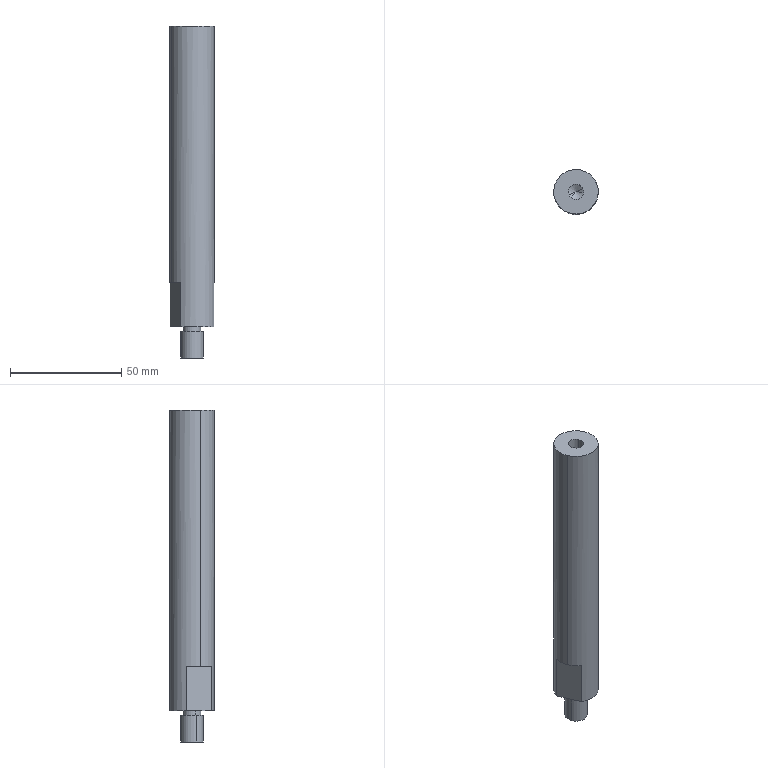Component | SolidWorks | -SmallSupport-2 | 1 solid | 18 faces | box 20 x 20 x 149 mm | volume 41968 mm3 | cylinder 8 | plane 8 | cone 2 | commonest cylinder face diameters 10 x2 8 x2 6.8 x2 20 x2
build123d program:
from build123d import *

# Parameters (mm, degrees)
SKETCH1_R             = 10
BOSS_EXTRUDE1_DEPTH   = 67.5
M8_TAPPED_HOLE1_D     = 6.8
M8_TAPPED_HOLE1_DEPTH = 22.25
M8_TAPPED_HOLE1_TIP   = 2.043
SKETCH4_R             = 4
BOSS_EXTRUDE2_DEPTH   = 2
SKETCH5_R             = 5
BOSS_EXTRUDE3_DEPTH   = 12
SKETCH6_W             = 8.326
SKETCH6_H             = 20.836
SKETCH6_W_2           = 8.024
SKETCH6_H_2           = 19.024
CUT_EXTRUDE1_DEPTH    = 20


with BuildPart() as part:
    # Sketch1 → Boss-Extrude1 (new, symmetric)
    with BuildSketch(Plane.XY):
        Circle(SKETCH1_R)
    extrude(amount=BOSS_EXTRUDE1_DEPTH, both=True)

    # M8 Tapped Hole1
    with Locations(Plane(origin=(0, 0, -67.5), x_dir=(1, 0, 0), z_dir=(0, 0, -1))):
        with Locations((0, 0)):
            Hole(M8_TAPPED_HOLE1_D / 2, depth=M8_TAPPED_HOLE1_DEPTH)
            with Locations((0, 0, -(M8_TAPPED_HOLE1_DEPTH + M8_TAPPED_HOLE1_TIP / 2))):  # 118° drill point
                Cone(0, M8_TAPPED_HOLE1_D / 2, M8_TAPPED_HOLE1_TIP, mode=Mode.SUBTRACT)

    # Sketch4 → Boss-Extrude2 (add)
    with BuildSketch(Plane.XY.offset(67.5)):
        Circle(SKETCH4_R)
    extrude(amount=BOSS_EXTRUDE2_DEPTH)

    # Sketch5 → Boss-Extrude3 (add)
    with BuildSketch(Plane.XY.offset(69.5)):
        Circle(SKETCH5_R)
    extrude(amount=BOSS_EXTRUDE3_DEPTH)

    # Sketch6 → Cut-Extrude1 (cut)
    with BuildSketch(Plane.XY.offset(67.5)):
        with Locations((-12.163, -0.5023)):
            Rectangle(SKETCH6_W, SKETCH6_H)
        with Locations((12.012, -1.408)):
            Rectangle(SKETCH6_W_2, SKETCH6_H_2)
    extrude(amount=-CUT_EXTRUDE1_DEPTH, mode=Mode.SUBTRACT)


solid = part.part

# Placed as in the assembly
solid = solid.moved(Location((115, 1079.5, 72.5), (-180, 0, 157.477)))
STEP:
#1=COLOUR_RGB('',0.7922,0.8196,0.9333);
#2=FILL_AREA_STYLE_COLOUR('',#1);
#3=FILL_AREA_STYLE('',(#2));
#4=SURFACE_STYLE_FILL_AREA(#3);
#5=SURFACE_SIDE_STYLE('',(#4));
#6=SURFACE_STYLE_USAGE(.BOTH.,#5);
#7=PRESENTATION_STYLE_ASSIGNMENT((#6));
#8=CARTESIAN_POINT('',(4.346,42.425,-0.3543));
#9=VERTEX_POINT('',#8);
#10=CARTESIAN_POINT('',(4.709,42.575,-0.3543));
#11=VERTEX_POINT('',#10);
#12=CARTESIAN_POINT('',(4.528,42.5,-0.3543));
#13=DIRECTION('',(0.,0.,-1.));
#14=DIRECTION('',(-0.9237,-0.383,0.));
#15=AXIS2_PLACEMENT_3D('',#12,#13,#14);
#16=CIRCLE('',#15,0.1969);
#17=EDGE_CURVE('',#9,#11,#16,.T.);
#18=ORIENTED_EDGE('',*,*,#17,.F.);
#19=CARTESIAN_POINT('',(4.346,42.425,0.1181));
#20=VERTEX_POINT('',#19);
#21=CARTESIAN_POINT('',(4.346,42.425,-0.3543));
#22=DIRECTION('',(0.,0.,1.));
#23=VECTOR('',#22,39.37);
#24=LINE('',#21,#23);
#25=EDGE_CURVE('',#9,#20,#24,.T.);
#26=ORIENTED_EDGE('',*,*,#25,.T.);
#27=CARTESIAN_POINT('',(4.709,42.575,0.1181));
#28=VERTEX_POINT('',#27);
#29=CARTESIAN_POINT('',(4.528,42.5,0.1181));
#30=DIRECTION('',(0.,0.,-1.));
#31=DIRECTION('',(-0.9237,-0.383,0.));
#32=AXIS2_PLACEMENT_3D('',#29,#30,#31);
#33=CIRCLE('',#32,0.1969);
#34=EDGE_CURVE('',#20,#28,#33,.T.);
#35=ORIENTED_EDGE('',*,*,#34,.T.);
#36=CARTESIAN_POINT('',(4.709,42.575,-0.3543));
#37=DIRECTION('',(0.,0.,1.));
#38=VECTOR('',#37,39.37);
#39=LINE('',#36,#38);
#40=EDGE_CURVE('',#11,#28,#39,.T.);
#41=ORIENTED_EDGE('',*,*,#40,.F.);
#42=EDGE_LOOP('',(#18,#26,#35,#41));
#43=FACE_OUTER_BOUND('',#42,.T.);
#44=CARTESIAN_POINT('',(4.528,42.5,-0.3543));
#45=DIRECTION('',(0.,0.,1.));
#46=DIRECTION('',(0.9237,0.383,0.));
#47=AXIS2_PLACEMENT_3D('',#44,#45,#46);
#48=CYLINDRICAL_SURFACE('',#47,0.1969);
#49=ADVANCED_FACE('',(#43),#48,.T.);
#50=CARTESIAN_POINT('',(4.382,42.44,0.1181));
#51=VERTEX_POINT('',#50);
#52=CARTESIAN_POINT('',(4.673,42.56,0.1181));
#53=VERTEX_POINT('',#52);
#54=CARTESIAN_POINT('',(4.528,42.5,0.1181));
#55=DIRECTION('',(0.,0.,-1.));
#56=DIRECTION('',(-0.9237,-0.383,0.));
#57=AXIS2_PLACEMENT_3D('',#54,#55,#56);
#58=CIRCLE('',#57,0.1575);
#59=EDGE_CURVE('',#51,#53,#58,.T.);
#60=ORIENTED_EDGE('',*,*,#59,.F.);
#61=CARTESIAN_POINT('',(4.382,42.44,0.1969));
#62=VERTEX_POINT('',#61);
#63=CARTESIAN_POINT('',(4.382,42.44,0.1181));
#64=DIRECTION('',(0.,0.,1.));
#65=VECTOR('',#64,39.37);
#66=LINE('',#63,#65);
#67=EDGE_CURVE('',#51,#62,#66,.T.);
#68=ORIENTED_EDGE('',*,*,#67,.T.);
#69=CARTESIAN_POINT('',(4.673,42.56,0.1969));
#70=VERTEX_POINT('',#69);
#71=CARTESIAN_POINT('',(4.528,42.5,0.1969));
#72=DIRECTION('',(0.,0.,-1.));
#73=DIRECTION('',(-0.9237,-0.383,0.));
#74=AXIS2_PLACEMENT_3D('',#71,#72,#73);
#75=CIRCLE('',#74,0.1575);
#76=EDGE_CURVE('',#62,#70,#75,.T.);
#77=ORIENTED_EDGE('',*,*,#76,.T.);
#78=CARTESIAN_POINT('',(4.673,42.56,0.1181));
#79=DIRECTION('',(0.,0.,1.));
#80=VECTOR('',#79,39.37);
#81=LINE('',#78,#80);
#82=EDGE_CURVE('',#53,#70,#81,.T.);
#83=ORIENTED_EDGE('',*,*,#82,.F.);
#84=EDGE_LOOP('',(#60,#68,#77,#83));
#85=FACE_OUTER_BOUND('',#84,.T.);
#86=CARTESIAN_POINT('',(4.528,42.5,0.1181));
#87=DIRECTION('',(0.,0.,1.));
#88=DIRECTION('',(0.9237,0.383,0.));
#89=AXIS2_PLACEMENT_3D('',#86,#87,#88);
#90=CYLINDRICAL_SURFACE('',#89,0.1575);
#91=ADVANCED_FACE('',(#85),#90,.T.);
#92=CARTESIAN_POINT('',(4.404,42.449,4.636));
#93=VERTEX_POINT('',#92);
#94=CARTESIAN_POINT('',(4.651,42.551,4.636));
#95=VERTEX_POINT('',#94);
#96=CARTESIAN_POINT('',(4.528,42.5,4.636));
#97=DIRECTION('',(0.,0.,1.));
#98=DIRECTION('',(0.9237,0.383,0.));
#99=AXIS2_PLACEMENT_3D('',#96,#97,#98);
#100=CIRCLE('',#99,0.1339);
#101=EDGE_CURVE('',#93,#95,#100,.T.);
#102=ORIENTED_EDGE('',*,*,#101,.F.);
#103=CARTESIAN_POINT('',(4.404,42.449,5.512));
#104=VERTEX_POINT('',#103);
#105=CARTESIAN_POINT('',(4.404,42.449,5.512));
#106=DIRECTION('',(0.,0.,1.));
#107=VECTOR('',#106,39.37);
#108=LINE('',#105,#107);
#109=EDGE_CURVE('',#93,#104,#108,.T.);
#110=ORIENTED_EDGE('',*,*,#109,.T.);
#111=CARTESIAN_POINT('',(4.651,42.551,5.512));
#112=VERTEX_POINT('',#111);
#113=CARTESIAN_POINT('',(4.528,42.5,5.512));
#114=DIRECTION('',(0.,0.,1.));
#115=DIRECTION('',(0.9237,0.383,0.));
#116=AXIS2_PLACEMENT_3D('',#113,#114,#115);
#117=CIRCLE('',#116,0.1339);
#118=EDGE_CURVE('',#104,#112,#117,.T.);
#119=ORIENTED_EDGE('',*,*,#118,.T.);
#120=CARTESIAN_POINT('',(4.651,42.551,5.512));
#121=DIRECTION('',(0.,0.,1.));
#122=VECTOR('',#121,39.37);
#123=LINE('',#120,#122);
#124=EDGE_CURVE('',#95,#112,#123,.T.);
#125=ORIENTED_EDGE('',*,*,#124,.F.);
#126=EDGE_LOOP('',(#102,#110,#119,#125));
#127=FACE_OUTER_BOUND('',#126,.T.);
#128=CARTESIAN_POINT('',(4.528,42.5,5.512));
#129=DIRECTION('',(0.,0.,1.));
#130=DIRECTION('',(0.9237,0.383,0.));
#131=AXIS2_PLACEMENT_3D('',#128,#129,#130);
#132=CYLINDRICAL_SURFACE('',#131,0.1339);
#133=ADVANCED_FACE('',(#127),#132,.F.);
#134=CARTESIAN_POINT('',(4.528,42.5,4.555));
#135=VERTEX_POINT('',#134);
#136=CARTESIAN_POINT('',(4.651,42.551,4.636));
#137=DIRECTION('',(0.7918,0.3283,0.515));
#138=VECTOR('',#137,39.37);
#139=LINE('',#136,#138);
#140=EDGE_CURVE('',#135,#95,#139,.T.);
#141=ORIENTED_EDGE('',*,*,#140,.F.);
#142=CARTESIAN_POINT('',(4.404,42.449,4.636));
#143=DIRECTION('',(-0.7918,-0.3283,0.515));
#144=VECTOR('',#143,39.37);
#145=LINE('',#142,#144);
#146=EDGE_CURVE('',#135,#93,#145,.T.);
#147=ORIENTED_EDGE('',*,*,#146,.T.);
#148=ORIENTED_EDGE('',*,*,#101,.T.);
#149=EDGE_LOOP('',(#141,#147,#148));
#150=FACE_OUTER_BOUND('',#149,.T.);
#151=CARTESIAN_POINT('',(4.528,42.5,4.636));
#152=DIRECTION('',(0.,0.,1.));
#153=DIRECTION('',(0.9237,0.383,0.));
#154=AXIS2_PLACEMENT_3D('',#151,#152,#153);
#155=CONICAL_SURFACE('',#154,0.1339,1.03);
#156=ADVANCED_FACE('',(#150),#155,.F.);
#157=CARTESIAN_POINT('',(4.146,42.598,0.9843));
#158=VERTEX_POINT('',#157);
#159=CARTESIAN_POINT('',(4.164,42.349,0.9843));
#160=VERTEX_POINT('',#159);
#161=CARTESIAN_POINT('',(4.528,42.5,0.9843));
#162=DIRECTION('',(0.,0.,1.));
#163=DIRECTION('',(0.9237,0.383,0.));
#164=AXIS2_PLACEMENT_3D('',#161,#162,#163);
#165=CIRCLE('',#164,0.3937);
#166=EDGE_CURVE('',#158,#160,#165,.T.);
#167=ORIENTED_EDGE('',*,*,#166,.T.);
#168=CARTESIAN_POINT('',(4.164,42.349,5.512));
#169=VERTEX_POINT('',#168);
#170=CARTESIAN_POINT('',(4.164,42.349,0.1969));
#171=DIRECTION('',(0.,0.,1.));
#172=VECTOR('',#171,39.37);
#173=LINE('',#170,#172);
#174=EDGE_CURVE('',#160,#169,#173,.T.);
#175=ORIENTED_EDGE('',*,*,#174,.T.);
#176=CARTESIAN_POINT('',(4.891,42.651,5.512));
#177=VERTEX_POINT('',#176);
#178=CARTESIAN_POINT('',(4.528,42.5,5.512));
#179=DIRECTION('',(0.,0.,-1.));
#180=DIRECTION('',(-0.9237,-0.383,0.));
#181=AXIS2_PLACEMENT_3D('',#178,#179,#180);
#182=CIRCLE('',#181,0.3937);
#183=EDGE_CURVE('',#169,#177,#182,.T.);
#184=ORIENTED_EDGE('',*,*,#183,.T.);
#185=CARTESIAN_POINT('',(4.891,42.651,0.9843));
#186=VERTEX_POINT('',#185);
#187=CARTESIAN_POINT('',(4.891,42.651,0.1969));
#188=DIRECTION('',(0.,0.,1.));
#189=VECTOR('',#188,39.37);
#190=LINE('',#187,#189);
#191=EDGE_CURVE('',#186,#177,#190,.T.);
#192=ORIENTED_EDGE('',*,*,#191,.F.);
#193=CARTESIAN_POINT('',(4.728,42.839,0.9843));
#194=VERTEX_POINT('',#193);
#195=CARTESIAN_POINT('',(4.528,42.5,0.9843));
#196=DIRECTION('',(0.,0.,-1.));
#197=DIRECTION('',(-0.9237,-0.383,0.));
#198=AXIS2_PLACEMENT_3D('',#195,#196,#197);
#199=CIRCLE('',#198,0.3937);
#200=EDGE_CURVE('',#194,#186,#199,.T.);
#201=ORIENTED_EDGE('',*,*,#200,.F.);
#202=CARTESIAN_POINT('',(4.728,42.839,0.1969));
#203=VERTEX_POINT('',#202);
#204=CARTESIAN_POINT('',(4.728,42.839,0.1969));
#205=DIRECTION('',(0.,0.,-1.));
#206=VECTOR('',#205,39.37);
#207=LINE('',#204,#206);
#208=EDGE_CURVE('',#194,#203,#207,.T.);
#209=ORIENTED_EDGE('',*,*,#208,.T.);
#210=CARTESIAN_POINT('',(4.146,42.598,0.1969));
#211=VERTEX_POINT('',#210);
#212=CARTESIAN_POINT('',(4.528,42.5,0.1969));
#213=DIRECTION('',(0.,0.,-1.));
#214=DIRECTION('',(-0.9237,-0.383,0.));
#215=AXIS2_PLACEMENT_3D('',#212,#213,#214);
#216=CIRCLE('',#215,0.3937);
#217=EDGE_CURVE('',#211,#203,#216,.T.);
#218=ORIENTED_EDGE('',*,*,#217,.F.);
#219=CARTESIAN_POINT('',(4.146,42.598,0.1969));
#220=DIRECTION('',(0.,0.,1.));
#221=VECTOR('',#220,39.37);
#222=LINE('',#219,#221);
#223=EDGE_CURVE('',#211,#158,#222,.T.);
#224=ORIENTED_EDGE('',*,*,#223,.T.);
#225=EDGE_LOOP('',(#167,#175,#184,#192,#201,#209,#218,#224));
#226=FACE_OUTER_BOUND('',#225,.T.);
#227=CARTESIAN_POINT('',(4.528,42.5,0.1969));
#228=DIRECTION('',(0.,0.,1.));
#229=DIRECTION('',(0.9237,0.383,0.));
#230=AXIS2_PLACEMENT_3D('',#227,#228,#229);
#231=CYLINDRICAL_SURFACE('',#230,0.3937);
#232=ADVANCED_FACE('',(#226),#231,.T.);
#233=CARTESIAN_POINT('',(4.327,42.161,0.1969));
#234=VERTEX_POINT('',#233);
#235=CARTESIAN_POINT('',(4.114,42.674,0.1969));
#236=DIRECTION('',(0.383,-0.9237,0.));
#237=VECTOR('',#236,39.37);
#238=LINE('',#235,#237);
#239=EDGE_CURVE('',#211,#234,#238,.T.);
#240=ORIENTED_EDGE('',*,*,#239,.F.);
#241=ORIENTED_EDGE('',*,*,#217,.T.);
#242=CARTESIAN_POINT('',(4.909,42.402,0.1969));
#243=VERTEX_POINT('',#242);
#244=CARTESIAN_POINT('',(4.669,42.981,0.1969));
#245=DIRECTION('',(-0.383,0.9237,0.));
#246=VECTOR('',#245,39.37);
#247=LINE('',#244,#246);
#248=EDGE_CURVE('',#243,#203,#247,.T.);
#249=ORIENTED_EDGE('',*,*,#248,.F.);
#250=CARTESIAN_POINT('',(4.528,42.5,0.1969));
#251=DIRECTION('',(0.,0.,-1.));
#252=DIRECTION('',(-0.9237,-0.383,0.));
#253=AXIS2_PLACEMENT_3D('',#250,#251,#252);
#254=CIRCLE('',#253,0.3937);
#255=EDGE_CURVE('',#243,#234,#254,.T.);
#256=ORIENTED_EDGE('',*,*,#255,.T.);
#257=EDGE_LOOP('',(#240,#241,#249,#256));
#258=FACE_OUTER_BOUND('',#257,.T.);
#259=CARTESIAN_POINT('',(4.528,42.5,0.1969));
#260=DIRECTION('',(0.,0.,-1.));
#261=DIRECTION('',(-0.9237,-0.383,0.));
#262=AXIS2_PLACEMENT_3D('',#259,#260,#261);
#263=CIRCLE('',#262,0.1575);
#264=EDGE_CURVE('',#70,#62,#263,.T.);
#265=ORIENTED_EDGE('',*,*,#264,.F.);
#266=ORIENTED_EDGE('',*,*,#76,.F.);
#267=EDGE_LOOP('',(#265,#266));
#268=FACE_BOUND('',#267,.T.);
#269=CARTESIAN_POINT('',(4.528,42.5,0.1969));
#270=DIRECTION('',(0.,0.,-1.));
#271=DIRECTION('',(-0.9237,-0.383,0.));
#272=AXIS2_PLACEMENT_3D('',#269,#270,#271);
#273=PLANE('',#272);
#274=ADVANCED_FACE('',(#258,#268),#273,.T.);
#275=ORIENTED_EDGE('',*,*,#174,.F.);
#276=CARTESIAN_POINT('',(4.327,42.161,0.9843));
#277=VERTEX_POINT('',#276);
#278=CARTESIAN_POINT('',(4.528,42.5,0.9843));
#279=DIRECTION('',(0.,0.,1.));
#280=DIRECTION('',(0.9237,0.383,0.));
#281=AXIS2_PLACEMENT_3D('',#278,#279,#280);
#282=CIRCLE('',#281,0.3937);
#283=EDGE_CURVE('',#160,#277,#282,.T.);
#284=ORIENTED_EDGE('',*,*,#283,.T.);
#285=CARTESIAN_POINT('',(4.327,42.161,0.1969));
#286=DIRECTION('',(0.,0.,-1.));
#287=VECTOR('',#286,39.37);
#288=LINE('',#285,#287);
#289=EDGE_CURVE('',#277,#234,#288,.T.);
#290=ORIENTED_EDGE('',*,*,#289,.T.);
#291=ORIENTED_EDGE('',*,*,#255,.F.);
#292=CARTESIAN_POINT('',(4.909,42.402,0.9843));
#293=VERTEX_POINT('',#292);
#294=CARTESIAN_POINT('',(4.909,42.402,0.1969));
#295=DIRECTION('',(0.,0.,1.));
#296=VECTOR('',#295,39.37);
#297=LINE('',#294,#296);
#298=EDGE_CURVE('',#243,#293,#297,.T.);
#299=ORIENTED_EDGE('',*,*,#298,.T.);
#300=CARTESIAN_POINT('',(4.528,42.5,0.9843));
#301=DIRECTION('',(0.,0.,-1.));
#302=DIRECTION('',(-0.9237,-0.383,0.));
#303=AXIS2_PLACEMENT_3D('',#300,#301,#302);
#304=CIRCLE('',#303,0.3937);
#305=EDGE_CURVE('',#186,#293,#304,.T.);
#306=ORIENTED_EDGE('',*,*,#305,.F.);
#307=ORIENTED_EDGE('',*,*,#191,.T.);
#308=CARTESIAN_POINT('',(4.528,42.5,5.512));
#309=DIRECTION('',(0.,0.,-1.));
#310=DIRECTION('',(-0.9237,-0.383,0.));
#311=AXIS2_PLACEMENT_3D('',#308,#309,#310);
#312=CIRCLE('',#311,0.3937);
#313=EDGE_CURVE('',#177,#169,#312,.T.);
#314=ORIENTED_EDGE('',*,*,#313,.T.);
#315=EDGE_LOOP('',(#275,#284,#290,#291,#299,#306,#307,#314));
#316=FACE_OUTER_BOUND('',#315,.T.);
#317=CARTESIAN_POINT('',(4.528,42.5,0.1969));
#318=DIRECTION('',(0.,0.,1.));
#319=DIRECTION('',(0.9237,0.383,0.));
#320=AXIS2_PLACEMENT_3D('',#317,#318,#319);
#321=CYLINDRICAL_SURFACE('',#320,0.3937);
#322=ADVANCED_FACE('',(#316),#321,.T.);
#323=CARTESIAN_POINT('',(4.528,42.5,5.512));
#324=DIRECTION('',(0.,0.,1.));
#325=DIRECTION('',(0.9237,0.383,0.));
#326=AXIS2_PLACEMENT_3D('',#323,#324,#325);
#327=CIRCLE('',#326,0.1339);
#328=EDGE_CURVE('',#112,#104,#327,.T.);
#329=ORIENTED_EDGE('',*,*,#328,.F.);
#330=ORIENTED_EDGE('',*,*,#118,.F.);
#331=EDGE_LOOP('',(#329,#330));
#332=FACE_BOUND('',#331,.T.);
#333=ORIENTED_EDGE('',*,*,#313,.F.);
#334=ORIENTED_EDGE('',*,*,#183,.F.);
#335=EDGE_LOOP('',(#333,#334));
#336=FACE_OUTER_BOUND('',#335,.T.);
#337=CARTESIAN_POINT('',(4.528,42.5,5.512));
#338=DIRECTION('',(0.,0.,-1.));
#339=DIRECTION('',(-0.9237,-0.383,0.));
#340=AXIS2_PLACEMENT_3D('',#337,#338,#339);
#341=PLANE('',#340);
#342=ADVANCED_FACE('',(#332,#336),#341,.F.);
#343=ORIENTED_EDGE('',*,*,#146,.F.);
#344=ORIENTED_EDGE('',*,*,#140,.T.);
#345=CARTESIAN_POINT('',(4.528,42.5,4.636));
#346=DIRECTION('',(0.,0.,1.));
#347=DIRECTION('',(0.9237,0.383,0.));
#348=AXIS2_PLACEMENT_3D('',#345,#346,#347);
#349=CIRCLE('',#348,0.1339);
#350=EDGE_CURVE('',#95,#93,#349,.T.);
#351=ORIENTED_EDGE('',*,*,#350,.T.);
#352=EDGE_LOOP('',(#343,#344,#351));
#353=FACE_OUTER_BOUND('',#352,.T.);
#354=CARTESIAN_POINT('',(4.528,42.5,4.636));
#355=DIRECTION('',(0.,0.,1.));
#356=DIRECTION('',(0.9237,0.383,0.));
#357=AXIS2_PLACEMENT_3D('',#354,#355,#356);
#358=CONICAL_SURFACE('',#357,0.1339,1.03);
#359=ADVANCED_FACE('',(#353),#358,.F.);
#360=ORIENTED_EDGE('',*,*,#109,.F.);
#361=ORIENTED_EDGE('',*,*,#350,.F.);
#362=ORIENTED_EDGE('',*,*,#124,.T.);
#363=ORIENTED_EDGE('',*,*,#328,.T.);
#364=EDGE_LOOP('',(#360,#361,#362,#363));
#365=FACE_OUTER_BOUND('',#364,.T.);
#366=CARTESIAN_POINT('',(4.528,42.5,5.512));
#367=DIRECTION('',(0.,0.,1.));
#368=DIRECTION('',(0.9237,0.383,0.));
#369=AXIS2_PLACEMENT_3D('',#366,#367,#368);
#370=CYLINDRICAL_SURFACE('',#369,0.1339);
#371=ADVANCED_FACE('',(#365),#370,.F.);
#372=ORIENTED_EDGE('',*,*,#67,.F.);
#373=CARTESIAN_POINT('',(4.528,42.5,0.1181));
#374=DIRECTION('',(0.,0.,-1.));
#375=DIRECTION('',(-0.9237,-0.383,0.));
#376=AXIS2_PLACEMENT_3D('',#373,#374,#375);
#377=CIRCLE('',#376,0.1575);
#378=EDGE_CURVE('',#53,#51,#377,.T.);
#379=ORIENTED_EDGE('',*,*,#378,.F.);
#380=ORIENTED_EDGE('',*,*,#82,.T.);
#381=ORIENTED_EDGE('',*,*,#264,.T.);
#382=EDGE_LOOP('',(#372,#379,#380,#381));
#383=FACE_OUTER_BOUND('',#382,.T.);
#384=CARTESIAN_POINT('',(4.528,42.5,0.1181));
#385=DIRECTION('',(0.,0.,1.));
#386=DIRECTION('',(0.9237,0.383,0.));
#387=AXIS2_PLACEMENT_3D('',#384,#385,#386);
#388=CYLINDRICAL_SURFACE('',#387,0.1575);
#389=ADVANCED_FACE('',(#383),#388,.T.);
#390=CARTESIAN_POINT('',(4.528,42.5,0.1181));
#391=DIRECTION('',(0.,0.,-1.));
#392=DIRECTION('',(-0.9237,-0.383,0.));
#393=AXIS2_PLACEMENT_3D('',#390,#391,#392);
#394=CIRCLE('',#393,0.1969);
#395=EDGE_CURVE('',#28,#20,#394,.T.);
#396=ORIENTED_EDGE('',*,*,#395,.F.);
#397=ORIENTED_EDGE('',*,*,#34,.F.);
#398=EDGE_LOOP('',(#396,#397));
#399=FACE_OUTER_BOUND('',#398,.T.);
#400=ORIENTED_EDGE('',*,*,#378,.T.);
#401=ORIENTED_EDGE('',*,*,#59,.T.);
#402=EDGE_LOOP('',(#400,#401));
#403=FACE_BOUND('',#402,.T.);
#404=CARTESIAN_POINT('',(4.528,42.5,0.1181));
#405=DIRECTION('',(0.,0.,-1.));
#406=DIRECTION('',(-0.9237,-0.383,0.));
#407=AXIS2_PLACEMENT_3D('',#404,#405,#406);
#408=PLANE('',#407);
#409=ADVANCED_FACE('',(#399,#403),#408,.F.);
#410=ORIENTED_EDGE('',*,*,#25,.F.);
#411=CARTESIAN_POINT('',(4.528,42.5,-0.3543));
#412=DIRECTION('',(0.,0.,-1.));
#413=DIRECTION('',(-0.9237,-0.383,0.));
#414=AXIS2_PLACEMENT_3D('',#411,#412,#413);
#415=CIRCLE('',#414,0.1969);
#416=EDGE_CURVE('',#11,#9,#415,.T.);
#417=ORIENTED_EDGE('',*,*,#416,.F.);
#418=ORIENTED_EDGE('',*,*,#40,.T.);
#419=ORIENTED_EDGE('',*,*,#395,.T.);
#420=EDGE_LOOP('',(#410,#417,#418,#419));
#421=FACE_OUTER_BOUND('',#420,.T.);
#422=CARTESIAN_POINT('',(4.528,42.5,-0.3543));
#423=DIRECTION('',(0.,0.,1.));
#424=DIRECTION('',(0.9237,0.383,0.));
#425=AXIS2_PLACEMENT_3D('',#422,#423,#424);
#426=CYLINDRICAL_SURFACE('',#425,0.1969);
#427=ADVANCED_FACE('',(#421),#426,.T.);
#428=ORIENTED_EDGE('',*,*,#416,.T.);
#429=ORIENTED_EDGE('',*,*,#17,.T.);
#430=EDGE_LOOP('',(#428,#429));
#431=FACE_OUTER_BOUND('',#430,.T.);
#432=CARTESIAN_POINT('',(4.528,42.5,-0.3543));
#433=DIRECTION('',(0.,0.,-1.));
#434=DIRECTION('',(-0.9237,-0.383,0.));
#435=AXIS2_PLACEMENT_3D('',#432,#433,#434);
#436=PLANE('',#435);
#437=ADVANCED_FACE('',(#431),#436,.T.);
#438=ORIENTED_EDGE('',*,*,#248,.T.);
#439=ORIENTED_EDGE('',*,*,#208,.F.);
#440=CARTESIAN_POINT('',(4.669,42.981,0.9843));
#441=DIRECTION('',(-0.383,0.9237,0.));
#442=VECTOR('',#441,39.37);
#443=LINE('',#440,#442);
#444=EDGE_CURVE('',#293,#194,#443,.T.);
#445=ORIENTED_EDGE('',*,*,#444,.F.);
#446=ORIENTED_EDGE('',*,*,#298,.F.);
#447=EDGE_LOOP('',(#438,#439,#445,#446));
#448=FACE_OUTER_BOUND('',#447,.T.);
#449=CARTESIAN_POINT('',(4.669,42.981,0.9843));
#450=DIRECTION('',(-0.9237,-0.383,0.));
#451=DIRECTION('',(-0.383,0.9237,0.));
#452=AXIS2_PLACEMENT_3D('',#449,#450,#451);
#453=PLANE('',#452);
#454=ADVANCED_FACE('',(#448),#453,.F.);
#455=ORIENTED_EDGE('',*,*,#200,.T.);
#456=ORIENTED_EDGE('',*,*,#305,.T.);
#457=ORIENTED_EDGE('',*,*,#444,.T.);
#458=EDGE_LOOP('',(#455,#456,#457));
#459=FACE_OUTER_BOUND('',#458,.T.);
#460=CARTESIAN_POINT('',(4.528,42.5,0.9843));
#461=DIRECTION('',(0.,0.,-1.));
#462=DIRECTION('',(-0.9237,-0.383,0.));
#463=AXIS2_PLACEMENT_3D('',#460,#461,#462);
#464=PLANE('',#463);
#465=ADVANCED_FACE('',(#459),#464,.T.);
#466=ORIENTED_EDGE('',*,*,#239,.T.);
#467=ORIENTED_EDGE('',*,*,#289,.F.);
#468=CARTESIAN_POINT('',(4.114,42.674,0.9843));
#469=DIRECTION('',(0.383,-0.9237,0.));
#470=VECTOR('',#469,39.37);
#471=LINE('',#468,#470);
#472=EDGE_CURVE('',#158,#277,#471,.T.);
#473=ORIENTED_EDGE('',*,*,#472,.F.);
#474=ORIENTED_EDGE('',*,*,#223,.F.);
#475=EDGE_LOOP('',(#466,#467,#473,#474));
#476=FACE_OUTER_BOUND('',#475,.T.);
#477=CARTESIAN_POINT('',(4.114,42.674,0.9843));
#478=DIRECTION('',(0.9237,0.383,0.));
#479=DIRECTION('',(0.383,-0.9237,0.));
#480=AXIS2_PLACEMENT_3D('',#477,#478,#479);
#481=PLANE('',#480);
#482=ADVANCED_FACE('',(#476),#481,.F.);
#483=ORIENTED_EDGE('',*,*,#472,.T.);
#484=ORIENTED_EDGE('',*,*,#283,.F.);
#485=ORIENTED_EDGE('',*,*,#166,.F.);
#486=EDGE_LOOP('',(#483,#484,#485));
#487=FACE_OUTER_BOUND('',#486,.T.);
#488=CARTESIAN_POINT('',(4.528,42.5,0.9843));
#489=DIRECTION('',(0.,0.,1.));
#490=DIRECTION('',(0.9237,0.383,0.));
#491=AXIS2_PLACEMENT_3D('',#488,#489,#490);
#492=PLANE('',#491);
#493=ADVANCED_FACE('',(#487),#492,.F.);
#494=CLOSED_SHELL('',(#49,#91,#133,#156,#232,#274,#322,#342,#359,#371,#389,#409,#427,#437,#454,#465,#482,#493));
#495=MANIFOLD_SOLID_BREP('',#494);
#496=STYLED_ITEM('',(#7),#495);
#497=(LENGTH_UNIT()NAMED_UNIT(*)SI_UNIT($,.METRE.));
#498=LENGTH_MEASURE_WITH_UNIT(LENGTH_MEASURE(0.0254),#497);
#499=DIMENSIONAL_EXPONENTS(1.,0.,0.,0.,0.,0.,0.);
#500=(CONVERSION_BASED_UNIT('',#498)LENGTH_UNIT()NAMED_UNIT(#499));
#501=UNCERTAINTY_MEASURE_WITH_UNIT(LENGTH_MEASURE(0.00001),#500,'','');
#502=(NAMED_UNIT(*)PLANE_ANGLE_UNIT()SI_UNIT($,.RADIAN.));
#503=(NAMED_UNIT(*)SI_UNIT($,.STERADIAN.)SOLID_ANGLE_UNIT());
#504=(GEOMETRIC_REPRESENTATION_CONTEXT(3)GLOBAL_UNCERTAINTY_ASSIGNED_CONTEXT((#501))GLOBAL_UNIT_ASSIGNED_CONTEXT((#500,#502,#503))REPRESENTATION_CONTEXT('',''));
#505=MECHANICAL_DESIGN_GEOMETRIC_PRESENTATION_REPRESENTATION('',(#496),#504);
#506=CARTESIAN_POINT('',(0.,0.,0.));
#507=DIRECTION('',(0.,0.,1.));
#508=DIRECTION('',(1.,0.,0.));
#509=AXIS2_PLACEMENT_3D('',#506,#507,#508);
#510=(LENGTH_UNIT()NAMED_UNIT(*)SI_UNIT($,.METRE.));
#511=LENGTH_MEASURE_WITH_UNIT(LENGTH_MEASURE(0.0254),#510);
#512=DIMENSIONAL_EXPONENTS(1.,0.,0.,0.,0.,0.,0.);
#513=(CONVERSION_BASED_UNIT('',#511)LENGTH_UNIT()NAMED_UNIT(#512));
#514=UNCERTAINTY_MEASURE_WITH_UNIT(LENGTH_MEASURE(0.00001),#513,'','');
#515=(NAMED_UNIT(*)PLANE_ANGLE_UNIT()SI_UNIT($,.RADIAN.));
#516=(NAMED_UNIT(*)SI_UNIT($,.STERADIAN.)SOLID_ANGLE_UNIT());
#517=(GEOMETRIC_REPRESENTATION_CONTEXT(3)GLOBAL_UNCERTAINTY_ASSIGNED_CONTEXT((#514))GLOBAL_UNIT_ASSIGNED_CONTEXT((#513,#515,#516))REPRESENTATION_CONTEXT('',''));
#518=ADVANCED_BREP_SHAPE_REPRESENTATION('',(#495,#509),#517);
#519=PRESENTATION_LAYER_ASSIGNMENT('','',(#496));